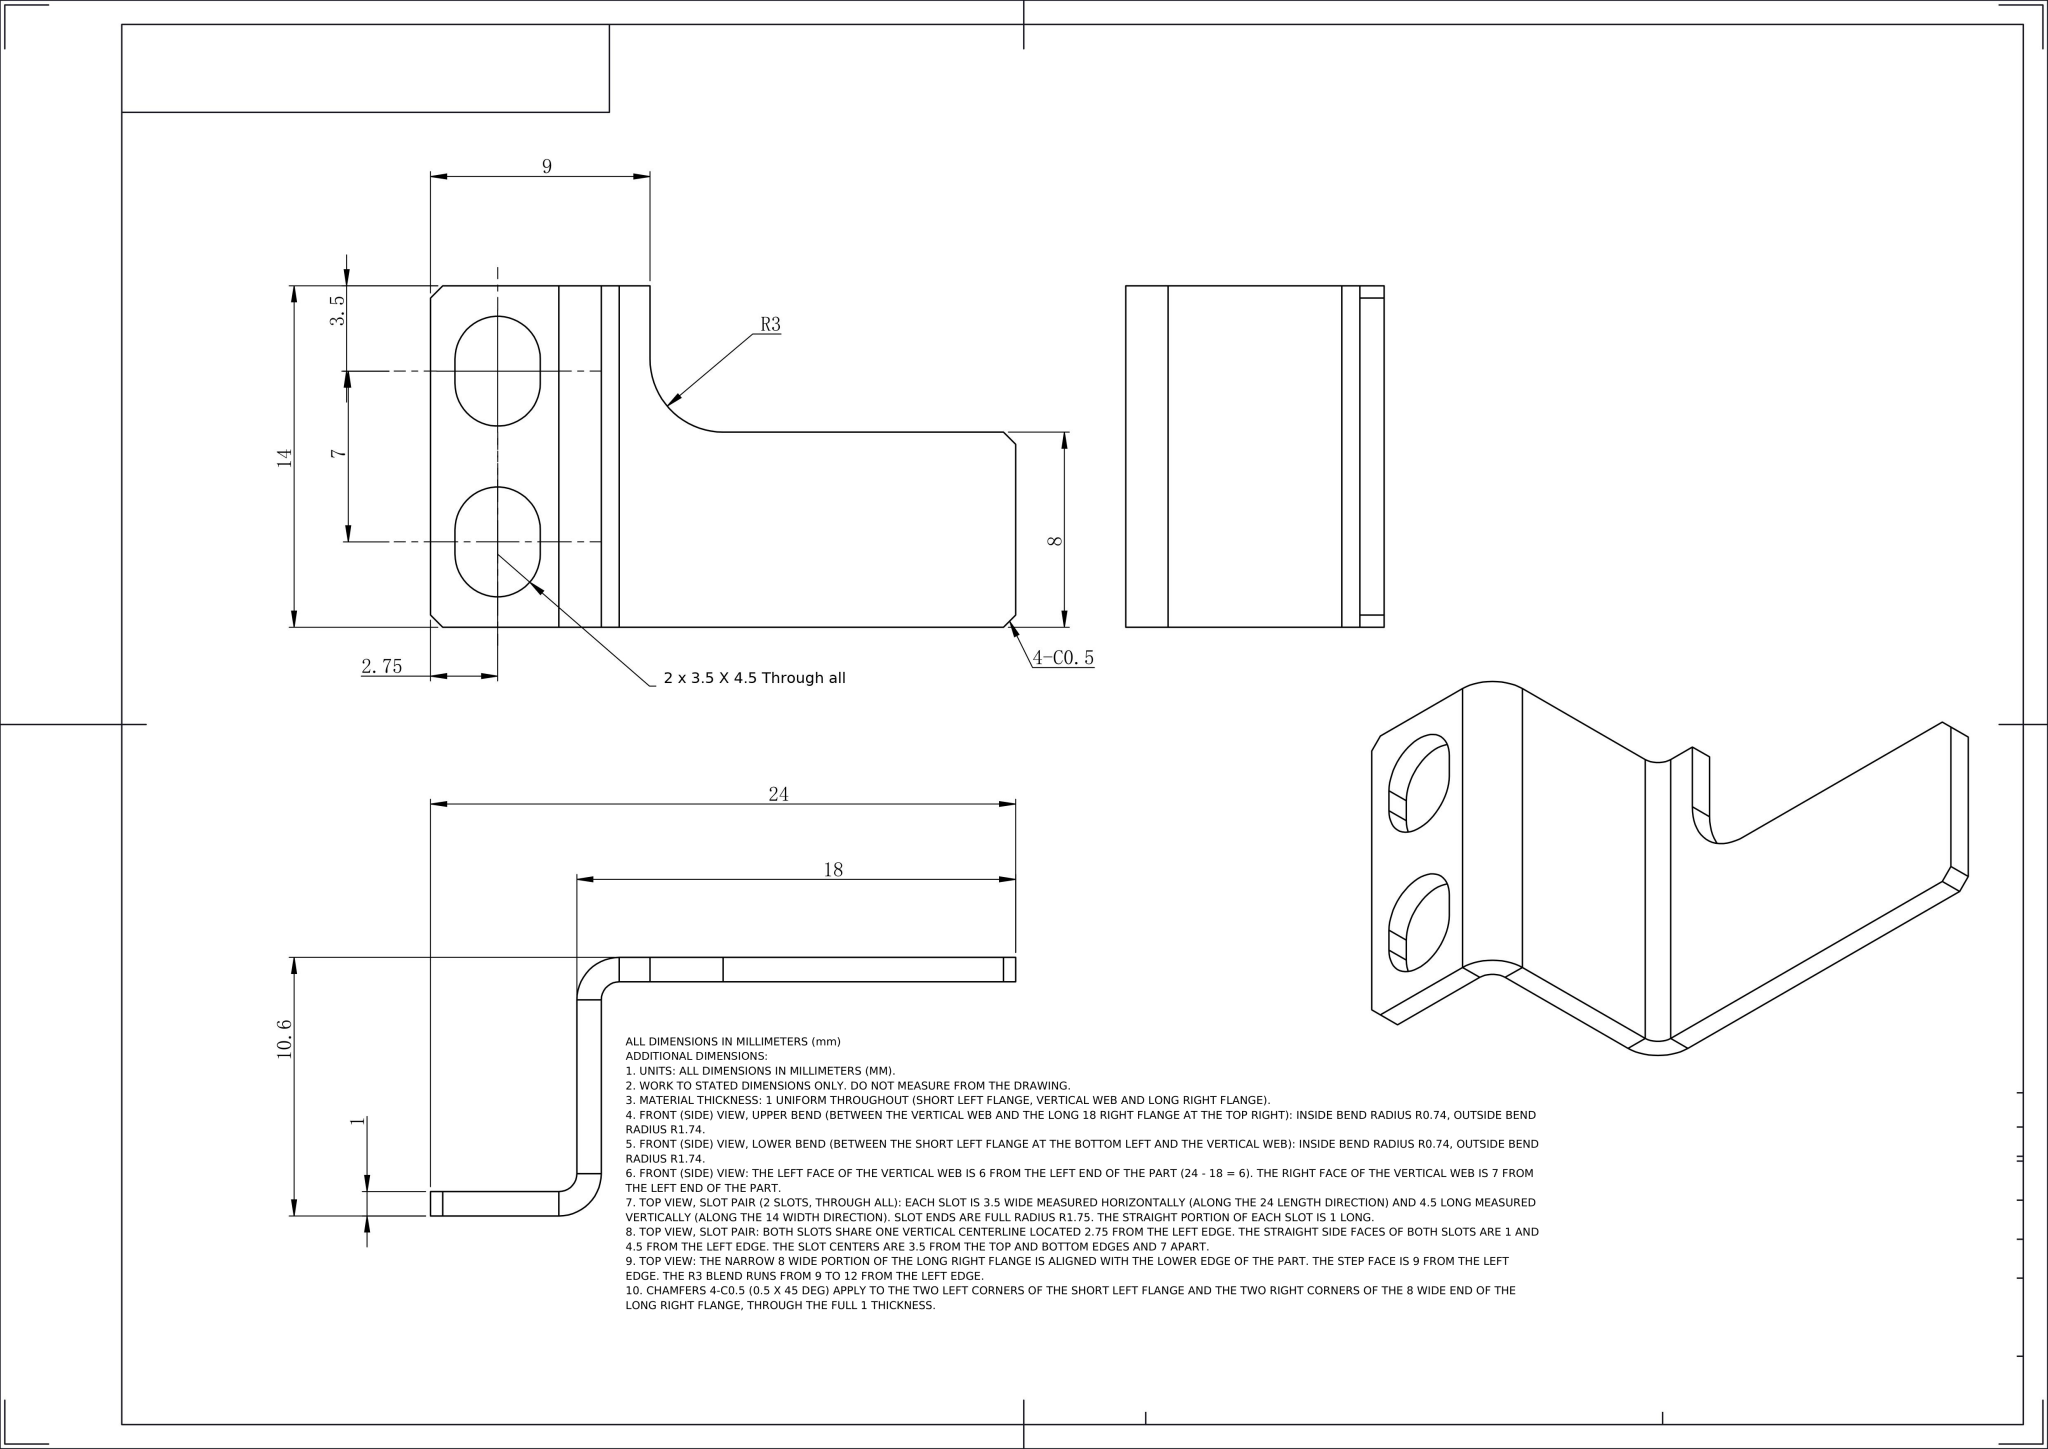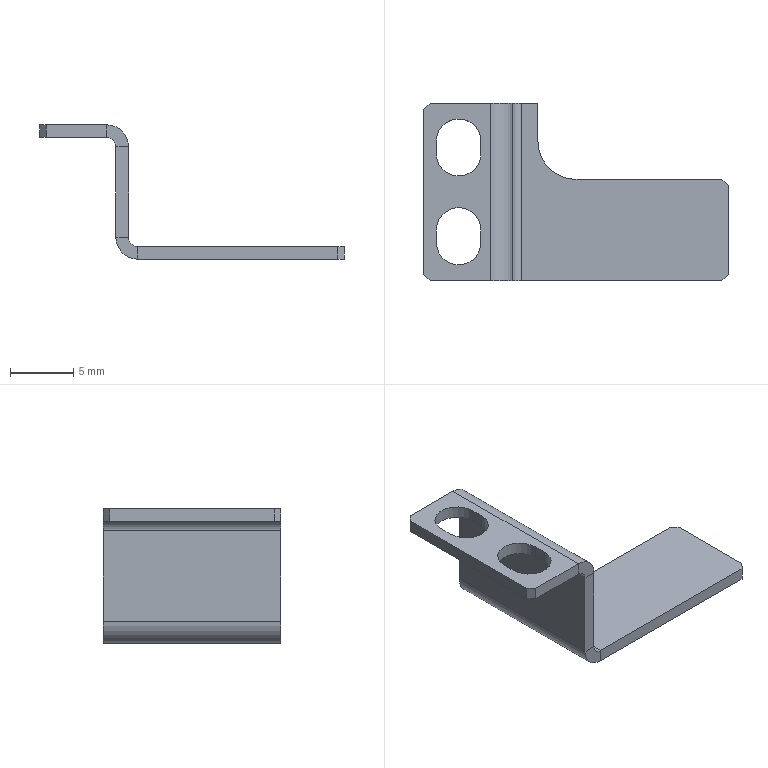Part | NX | mm | 1 solid | 37 faces | box 24 x 14 x 10.6 mm | volume 341 mm3 | plane 28 | cylinder 9 | commonest cylinder face diameters 3.5 x4 3.473 x2 1.473 x2 6 x1